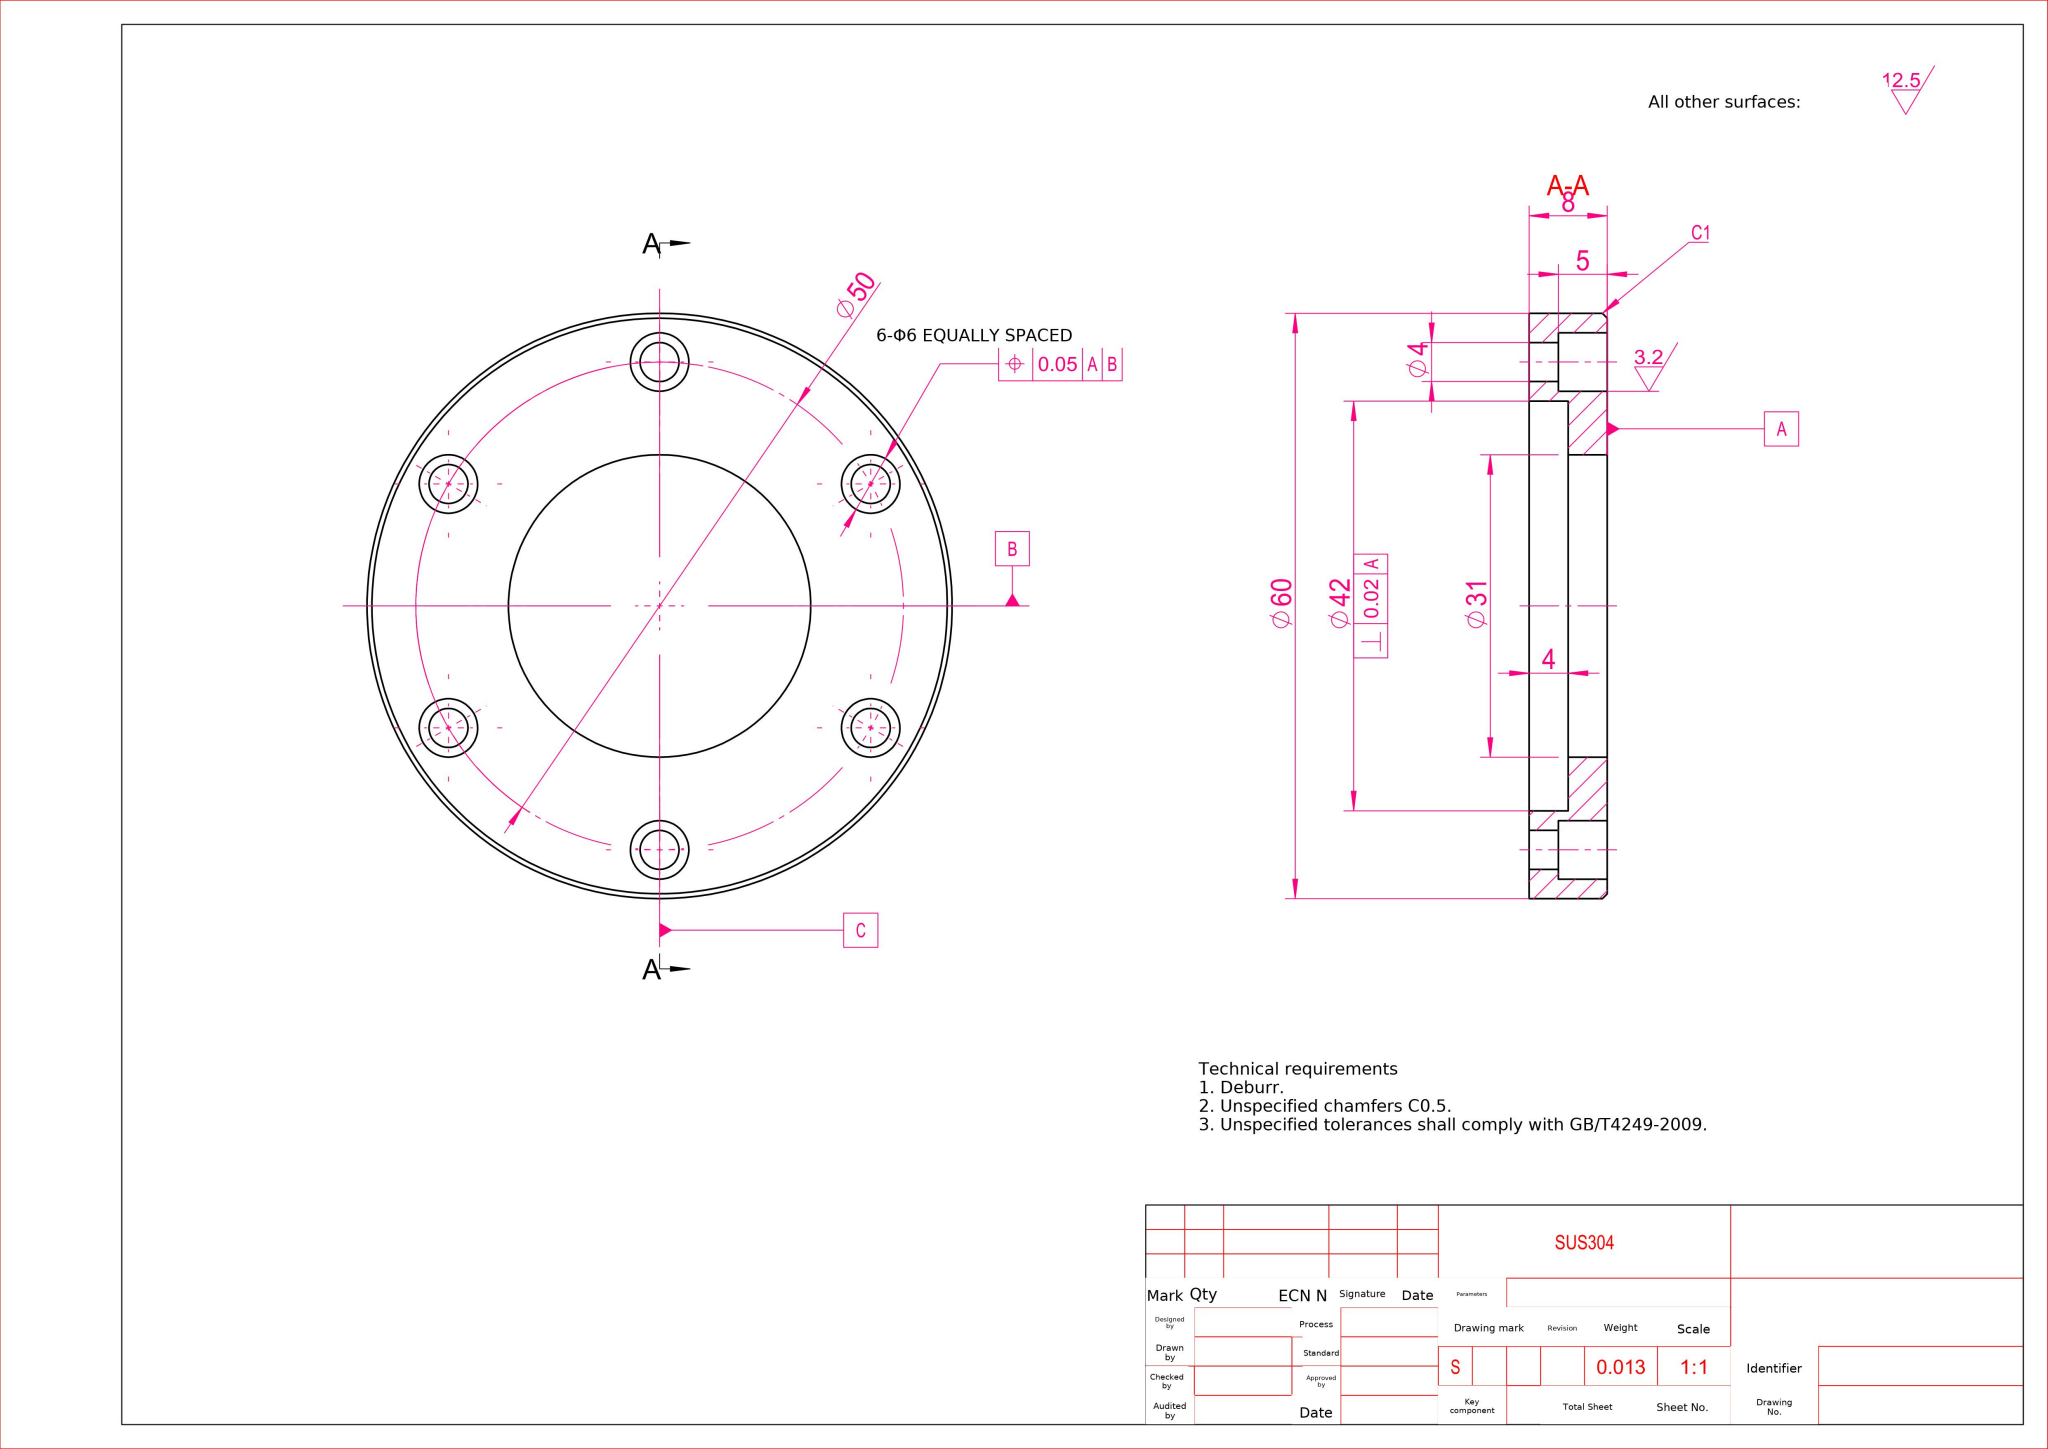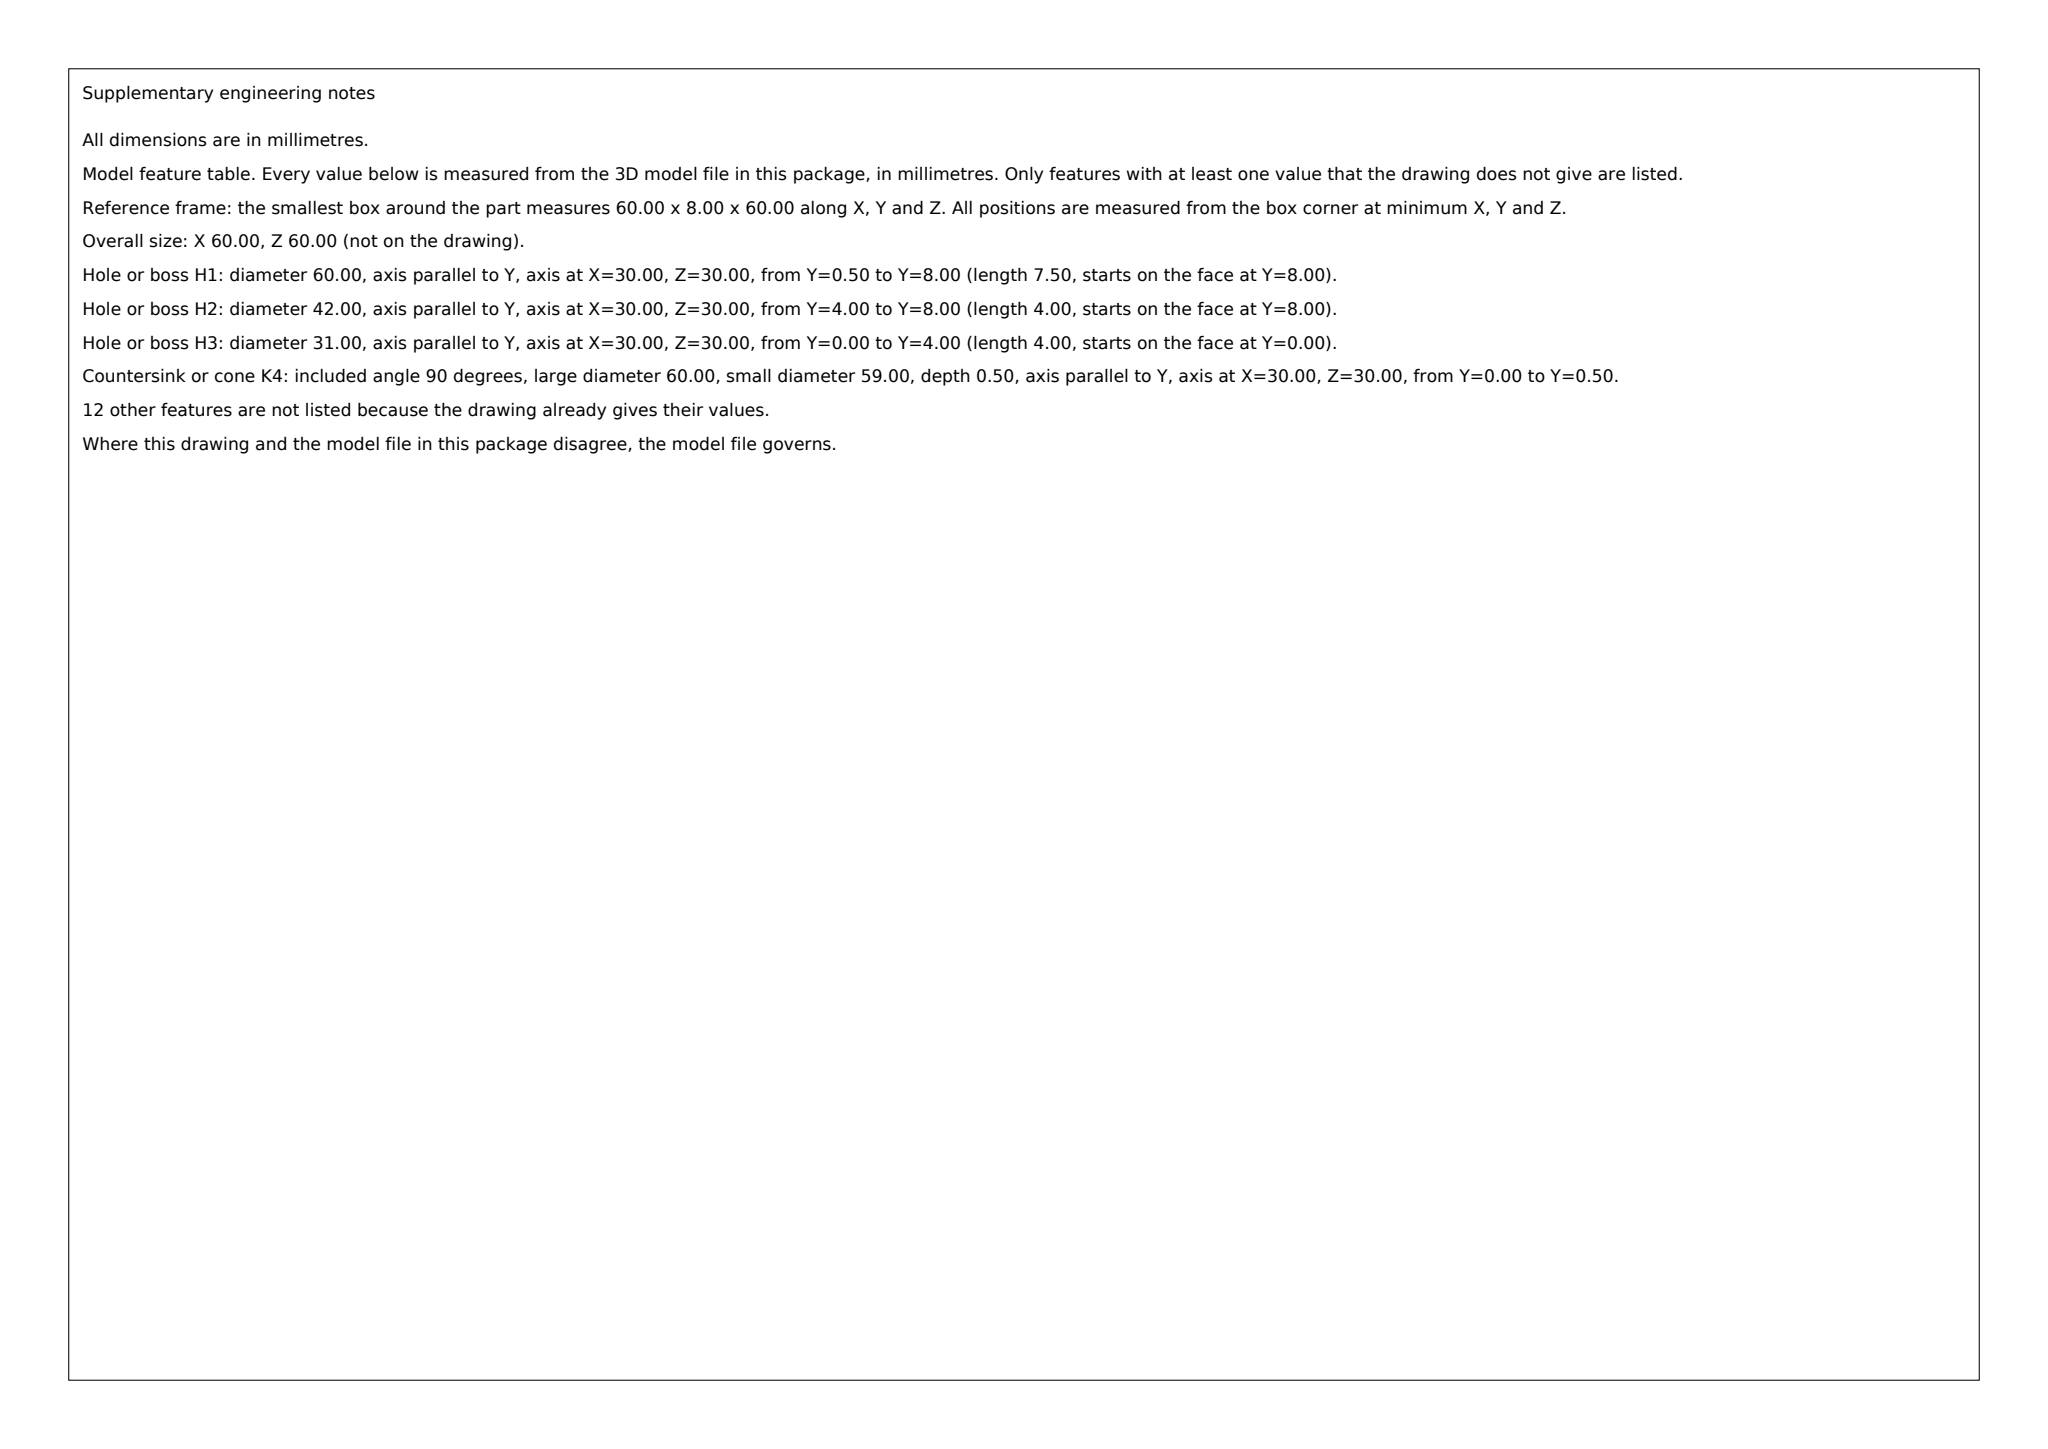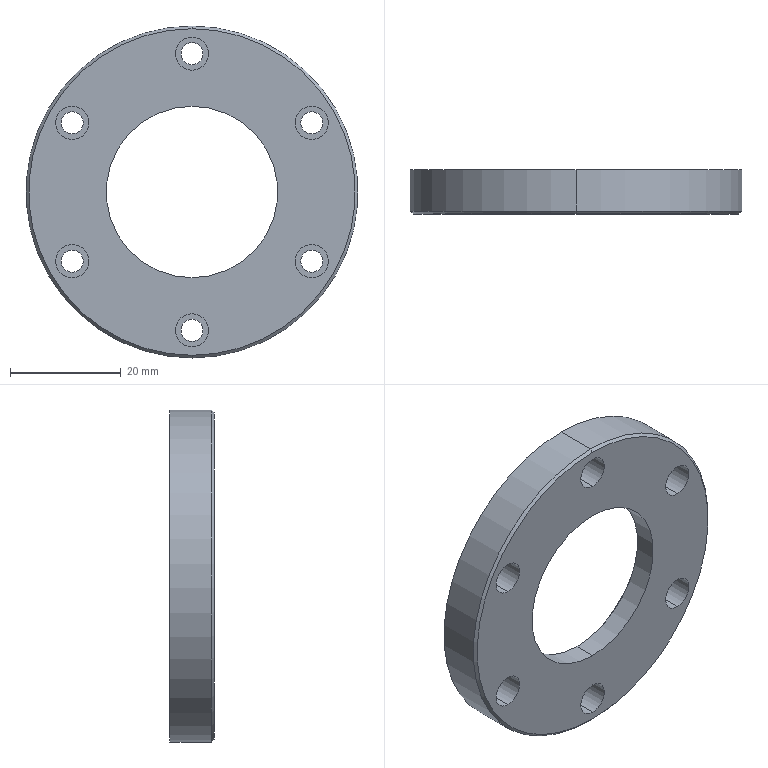Part | SolidWorks | mm | material SUS304 | 1 solid | 41 faces | box 60 x 8 x 60 mm | volume 12961 mm3 | cylinder 30 | plane 9 | cone 2 | commonest cylinder face diameters 6 x12 4 x12 42 x2 60 x2 31 x2
build123d program:
from build123d import *

# Parameters (mm, degrees)
SKETCH1_R                      = 30
SKETCH1_R_2                    = 15.5
BOSS_EXTRUDE1_DEPTH            = 8
SKETCH2_R                      = 21
CUT_EXTRUDE1_DEPTH             = 4
CHAMFER1_SIZE                  = 0.5
F_4_0MM_DOWEL_PIN_HOLE_1_D     = 4
F_4_0MM_DOWEL_PIN_HOLE_1_DEPTH = 8
SKETCH7_R                      = 3
CUT_EXTRUDE3_DEPTH             = 5


with BuildPart() as part:
    # Sketch1 → Boss-Extrude1 (new body)
    with BuildSketch(Plane(origin=(0, 0, 0), x_dir=(1, 0, 0), z_dir=(0, 1, 0))):
        with Locations(Location((0, 0, 0), (0, 0, 270))):
            Circle(SKETCH1_R)
        with Locations(Location((0, 0, 0), (0, 0, 270))):
            Circle(SKETCH1_R_2, mode=Mode.SUBTRACT)
    extrude(amount=BOSS_EXTRUDE1_DEPTH)

    # Sketch2 → Cut-Extrude1 (cut)
    with BuildSketch(Plane(origin=(0, 8, 0), x_dir=(1, 0, 0), z_dir=(0, 1, 0))):
        with Locations(Location((0, 0, 0), (0, 0, 270))):
            Circle(SKETCH2_R)
    extrude(amount=-CUT_EXTRUDE1_DEPTH, mode=Mode.SUBTRACT)

    # Chamfer1
    chamfer1_edges = [part.edges().sort_by_distance(p)[0] for p in [
        (0, 0, -30),
    ]]
    chamfer(chamfer1_edges, length=CHAMFER1_SIZE)

    # 4.0mm Dowel Pin Hole 1
    with Locations(Plane(origin=(0, 0, 0), x_dir=(-1, 0, 0), z_dir=(0, -1, 0))):
        with Locations((0, -25), (-21.651, -12.5), (-21.651, 12.5), (0, 25), (21.651, 12.5), (21.651, -12.5), (0, 0)):
            Hole(F_4_0MM_DOWEL_PIN_HOLE_1_D / 2, depth=F_4_0MM_DOWEL_PIN_HOLE_1_DEPTH)

    # Sketch7 → Cut-Extrude3 (cut)
    with BuildSketch(Plane.XZ):
        with Locations(Location((-21.651, 12.5, 0), (0, 0, 270))):
            Circle(SKETCH7_R)
        with Locations(Location((0, 25, 0), (0, 0, 270))):
            Circle(SKETCH7_R)
        with Locations(Location((21.651, 12.5, 0), (0, 0, 270))):
            Circle(SKETCH7_R)
        with Locations(Location((21.651, -12.5, 0), (0, 0, 270))):
            Circle(SKETCH7_R)
        with Locations(Location((0, -25, 0), (0, 0, 270))):
            Circle(SKETCH7_R)
        with Locations(Location((-21.651, -12.5, 0), (0, 0, 270))):
            Circle(SKETCH7_R)
    extrude(amount=-CUT_EXTRUDE3_DEPTH, mode=Mode.SUBTRACT)


solid = part.part